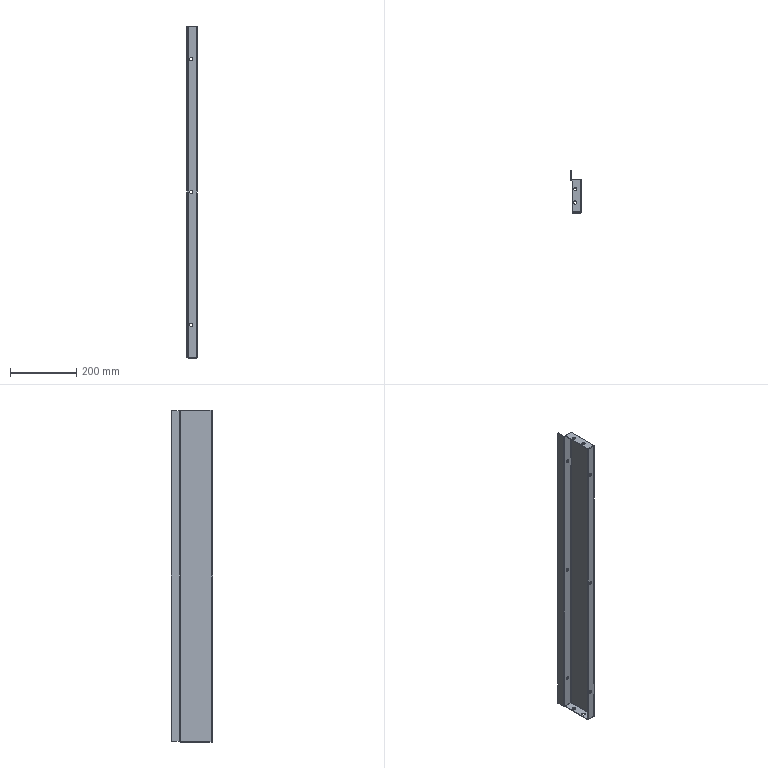Component | SolidWorks | 23BaseRightSidePlate-1 | 1 solid | 66 faces | volume 364167 mm3 | cylinder 30 | plane 28 | spline 8 | commonest cylinder face diameters 10 x20 2 x5 6 x5